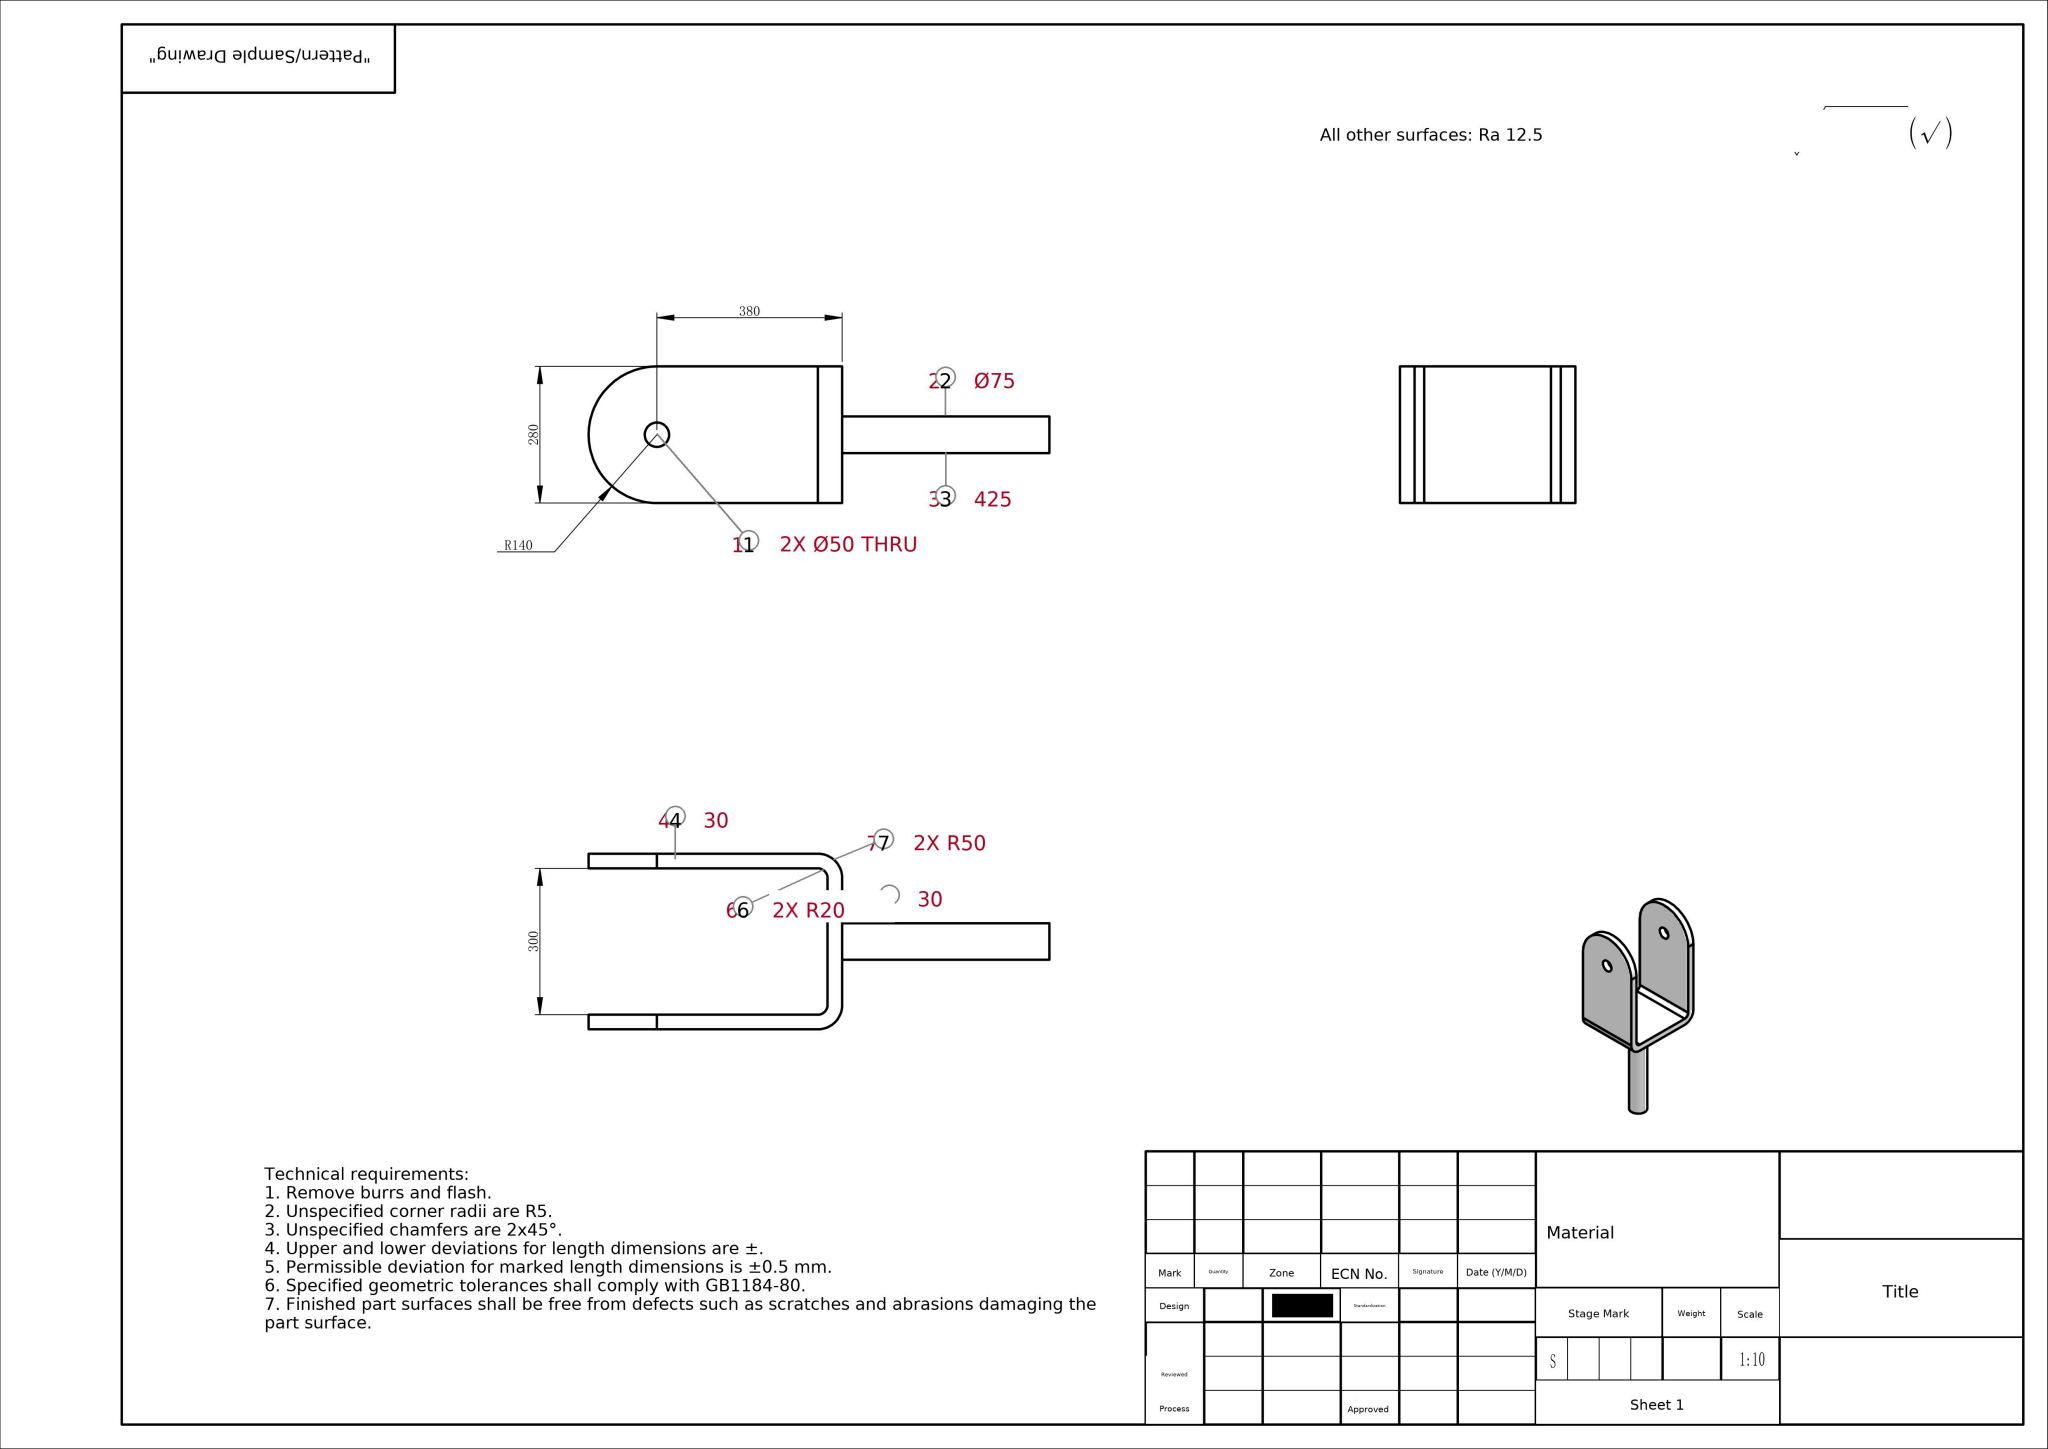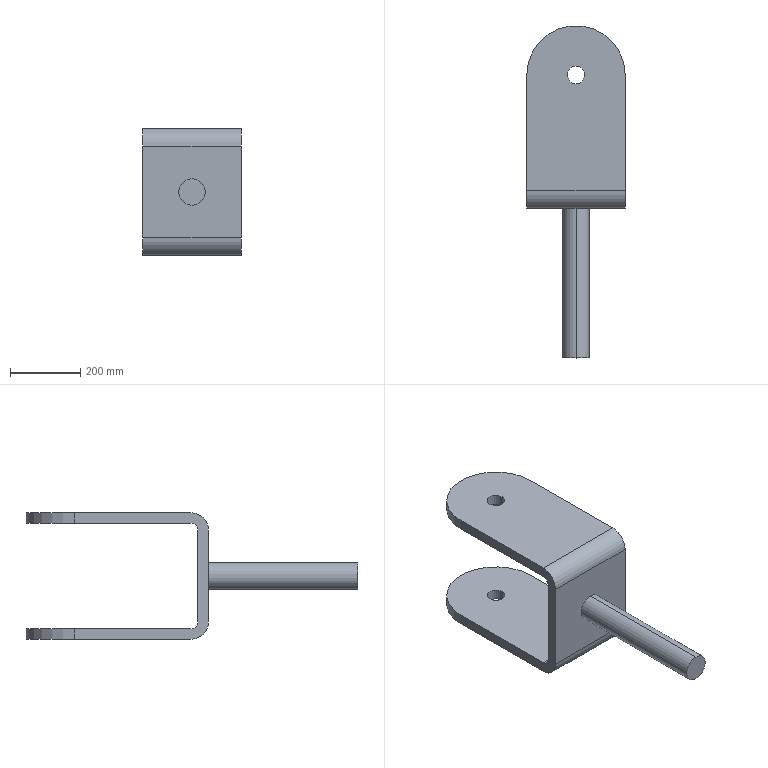Part | SolidWorks | mm | 1 solid | 21 faces | box 280 x 945 x 360 mm | volume 12258667 mm3 | cylinder 12 | plane 9 | commonest cylinder face diameters 50 x4 75 x2 280 x2 40 x2 100 x2
build123d program:
from build123d import *

# Parameters (mm, degrees)
SKETCH1_R           = 25
BOSS_EXTRUDE1_DEPTH = 360
SKETCH2_W           = 300
SKETCH2_H           = 490
CUT_EXTRUDE2_DEPTH  = 360
FILLET1_R           = 20
FILLET2_R           = 50
SKETCH3_R           = 37.5
BOSS_EXTRUDE2_DEPTH = 425


with BuildPart() as part:
    # Sketch1 → Boss-Extrude1 (new body)
    with BuildSketch(Plane.XY):
        with BuildLine():
            Line((-140, 0), (-140, -380))
            Line((-140, -380), (140, -380))
            Line((140, -380), (140, 0))
            ThreePointArc((140, 0), (0, 140), (-140, 0))
        make_face()
        with Locations(Location((0, 0, 0), (0, 0, 180))):
            Circle(SKETCH1_R, mode=Mode.SUBTRACT)
    extrude(amount=BOSS_EXTRUDE1_DEPTH)

    # Sketch2 → Cut-Extrude2 (cut)
    with BuildSketch(Plane(origin=(140, 0, 0), x_dir=(0, 0, -1), z_dir=(1, 0, 0))):
        with Locations((-180, -105)):
            Rectangle(SKETCH2_W, SKETCH2_H)
    extrude(amount=-CUT_EXTRUDE2_DEPTH, mode=Mode.SUBTRACT)

    # Fillet1
    fillet1_edges = [part.edges().sort_by_distance(p)[0] for p in [
        (0, -350, 30),
        (0, -350, 330),
    ]]
    fillet(fillet1_edges, radius=FILLET1_R)

    # Fillet2
    fillet2_edges = [part.edges().sort_by_distance(p)[0] for p in [
        (0, -380, 360),
        (0, -380, 0),
    ]]
    fillet(fillet2_edges, radius=FILLET2_R)

    # Sketch3 → Boss-Extrude2 (add)
    with BuildSketch(Plane.XZ.offset(380)):
        with Locations(Location((0, 180, 0), (0, 0, 90))):
            Circle(SKETCH3_R)
    extrude(amount=BOSS_EXTRUDE2_DEPTH)


solid = part.part
STEP:
#1=CARTESIAN_POINT('',(0.,-805.,142.5));
#2=VERTEX_POINT('',#1);
#3=CARTESIAN_POINT('',(0.,-805.,217.5));
#4=VERTEX_POINT('',#3);
#5=CARTESIAN_POINT('',(0.,-805.,180.));
#6=DIRECTION('',(0.,-1.,0.));
#7=DIRECTION('',(0.,0.,-1.));
#8=AXIS2_PLACEMENT_3D('',#5,#6,#7);
#9=CIRCLE('',#8,37.5);
#10=EDGE_CURVE('',#2,#4,#9,.T.);
#11=ORIENTED_EDGE('',*,*,#10,.F.);
#12=CARTESIAN_POINT('',(0.,-380.,142.5));
#13=VERTEX_POINT('',#12);
#14=CARTESIAN_POINT('',(0.,-805.,142.5));
#15=DIRECTION('',(0.,1.,0.));
#16=VECTOR('',#15,1000.);
#17=LINE('',#14,#16);
#18=EDGE_CURVE('',#2,#13,#17,.T.);
#19=ORIENTED_EDGE('',*,*,#18,.T.);
#20=CARTESIAN_POINT('',(0.,-380.,217.5));
#21=VERTEX_POINT('',#20);
#22=CARTESIAN_POINT('',(0.,-380.,180.));
#23=DIRECTION('',(0.,-1.,0.));
#24=DIRECTION('',(0.,0.,1.));
#25=AXIS2_PLACEMENT_3D('',#22,#23,#24);
#26=CIRCLE('',#25,37.5);
#27=EDGE_CURVE('',#13,#21,#26,.T.);
#28=ORIENTED_EDGE('',*,*,#27,.T.);
#29=CARTESIAN_POINT('',(0.,-805.,217.5));
#30=DIRECTION('',(0.,1.,0.));
#31=VECTOR('',#30,1000.);
#32=LINE('',#29,#31);
#33=EDGE_CURVE('',#4,#21,#32,.T.);
#34=ORIENTED_EDGE('',*,*,#33,.F.);
#35=EDGE_LOOP('',(#11,#19,#28,#34));
#36=FACE_OUTER_BOUND('',#35,.T.);
#37=CARTESIAN_POINT('',(0.,-805.,180.));
#38=DIRECTION('',(0.,1.,0.));
#39=DIRECTION('',(0.,0.,1.));
#40=AXIS2_PLACEMENT_3D('',#37,#38,#39);
#41=CYLINDRICAL_SURFACE('',#40,37.5);
#42=ADVANCED_FACE('',(#36),#41,.T.);
#43=CARTESIAN_POINT('',(-25.,0.,360.));
#44=VERTEX_POINT('',#43);
#45=CARTESIAN_POINT('',(25.,0.,360.));
#46=VERTEX_POINT('',#45);
#47=CARTESIAN_POINT('',(0.,0.,360.));
#48=DIRECTION('',(0.,0.,1.));
#49=DIRECTION('',(1.,0.,0.));
#50=AXIS2_PLACEMENT_3D('',#47,#48,#49);
#51=CIRCLE('',#50,25.);
#52=EDGE_CURVE('',#44,#46,#51,.T.);
#53=ORIENTED_EDGE('',*,*,#52,.T.);
#54=CARTESIAN_POINT('',(25.,0.,330.));
#55=VERTEX_POINT('',#54);
#56=CARTESIAN_POINT('',(25.,0.,360.));
#57=DIRECTION('',(0.,0.,-1.));
#58=VECTOR('',#57,1000.);
#59=LINE('',#56,#58);
#60=EDGE_CURVE('',#46,#55,#59,.T.);
#61=ORIENTED_EDGE('',*,*,#60,.T.);
#62=CARTESIAN_POINT('',(-25.,0.,330.));
#63=VERTEX_POINT('',#62);
#64=CARTESIAN_POINT('',(0.,0.,330.));
#65=DIRECTION('',(-0.,-0.,1.));
#66=DIRECTION('',(0.,-1.,0.));
#67=AXIS2_PLACEMENT_3D('',#64,#65,#66);
#68=CIRCLE('',#67,25.);
#69=EDGE_CURVE('',#63,#55,#68,.T.);
#70=ORIENTED_EDGE('',*,*,#69,.F.);
#71=CARTESIAN_POINT('',(-25.,0.,360.));
#72=DIRECTION('',(0.,0.,-1.));
#73=VECTOR('',#72,1000.);
#74=LINE('',#71,#73);
#75=EDGE_CURVE('',#44,#63,#74,.T.);
#76=ORIENTED_EDGE('',*,*,#75,.F.);
#77=EDGE_LOOP('',(#53,#61,#70,#76));
#78=FACE_OUTER_BOUND('',#77,.T.);
#79=CARTESIAN_POINT('',(0.,0.,360.));
#80=DIRECTION('',(0.,0.,-1.));
#81=DIRECTION('',(-1.,0.,0.));
#82=AXIS2_PLACEMENT_3D('',#79,#80,#81);
#83=CYLINDRICAL_SURFACE('',#82,25.);
#84=ADVANCED_FACE('',(#78),#83,.F.);
#85=CARTESIAN_POINT('',(25.,0.,30.));
#86=VERTEX_POINT('',#85);
#87=CARTESIAN_POINT('',(-25.,0.,30.));
#88=VERTEX_POINT('',#87);
#89=CARTESIAN_POINT('',(0.,0.,30.));
#90=DIRECTION('',(-0.,-0.,-1.));
#91=DIRECTION('',(0.,1.,0.));
#92=AXIS2_PLACEMENT_3D('',#89,#90,#91);
#93=CIRCLE('',#92,25.);
#94=EDGE_CURVE('',#86,#88,#93,.T.);
#95=ORIENTED_EDGE('',*,*,#94,.F.);
#96=CARTESIAN_POINT('',(25.,0.,0.));
#97=VERTEX_POINT('',#96);
#98=CARTESIAN_POINT('',(25.,0.,360.));
#99=DIRECTION('',(0.,0.,-1.));
#100=VECTOR('',#99,1000.);
#101=LINE('',#98,#100);
#102=EDGE_CURVE('',#86,#97,#101,.T.);
#103=ORIENTED_EDGE('',*,*,#102,.T.);
#104=CARTESIAN_POINT('',(-25.,0.,0.));
#105=VERTEX_POINT('',#104);
#106=CARTESIAN_POINT('',(0.,0.,0.));
#107=DIRECTION('',(0.,0.,1.));
#108=DIRECTION('',(1.,0.,0.));
#109=AXIS2_PLACEMENT_3D('',#106,#107,#108);
#110=CIRCLE('',#109,25.);
#111=EDGE_CURVE('',#105,#97,#110,.T.);
#112=ORIENTED_EDGE('',*,*,#111,.F.);
#113=CARTESIAN_POINT('',(-25.,0.,360.));
#114=DIRECTION('',(0.,0.,-1.));
#115=VECTOR('',#114,1000.);
#116=LINE('',#113,#115);
#117=EDGE_CURVE('',#88,#105,#116,.T.);
#118=ORIENTED_EDGE('',*,*,#117,.F.);
#119=EDGE_LOOP('',(#95,#103,#112,#118));
#120=FACE_OUTER_BOUND('',#119,.T.);
#121=CARTESIAN_POINT('',(0.,0.,360.));
#122=DIRECTION('',(0.,0.,-1.));
#123=DIRECTION('',(-1.,0.,0.));
#124=AXIS2_PLACEMENT_3D('',#121,#122,#123);
#125=CYLINDRICAL_SURFACE('',#124,25.);
#126=ADVANCED_FACE('',(#120),#125,.F.);
#127=CARTESIAN_POINT('',(-140.,-0.,30.));
#128=VERTEX_POINT('',#127);
#129=CARTESIAN_POINT('',(140.,0.,30.));
#130=VERTEX_POINT('',#129);
#131=CARTESIAN_POINT('',(0.,0.,30.));
#132=DIRECTION('',(-0.,-0.,-1.));
#133=DIRECTION('',(0.,1.,-0.));
#134=AXIS2_PLACEMENT_3D('',#131,#132,#133);
#135=CIRCLE('',#134,140.);
#136=EDGE_CURVE('',#128,#130,#135,.T.);
#137=ORIENTED_EDGE('',*,*,#136,.T.);
#138=CARTESIAN_POINT('',(140.,0.,0.));
#139=VERTEX_POINT('',#138);
#140=CARTESIAN_POINT('',(140.,0.,360.));
#141=DIRECTION('',(0.,0.,-1.));
#142=VECTOR('',#141,1000.);
#143=LINE('',#140,#142);
#144=EDGE_CURVE('',#130,#139,#143,.T.);
#145=ORIENTED_EDGE('',*,*,#144,.T.);
#146=CARTESIAN_POINT('',(-140.,0.,0.));
#147=VERTEX_POINT('',#146);
#148=CARTESIAN_POINT('',(0.,0.,0.));
#149=DIRECTION('',(0.,0.,1.));
#150=DIRECTION('',(1.,0.,0.));
#151=AXIS2_PLACEMENT_3D('',#148,#149,#150);
#152=CIRCLE('',#151,140.);
#153=EDGE_CURVE('',#139,#147,#152,.T.);
#154=ORIENTED_EDGE('',*,*,#153,.T.);
#155=CARTESIAN_POINT('',(-140.,0.,360.));
#156=DIRECTION('',(0.,0.,-1.));
#157=VECTOR('',#156,1000.);
#158=LINE('',#155,#157);
#159=EDGE_CURVE('',#128,#147,#158,.T.);
#160=ORIENTED_EDGE('',*,*,#159,.F.);
#161=EDGE_LOOP('',(#137,#145,#154,#160));
#162=FACE_OUTER_BOUND('',#161,.T.);
#163=CARTESIAN_POINT('',(0.,0.,360.));
#164=DIRECTION('',(0.,0.,-1.));
#165=DIRECTION('',(-1.,0.,0.));
#166=AXIS2_PLACEMENT_3D('',#163,#164,#165);
#167=CYLINDRICAL_SURFACE('',#166,140.);
#168=ADVANCED_FACE('',(#162),#167,.T.);
#169=ORIENTED_EDGE('',*,*,#102,.F.);
#170=CARTESIAN_POINT('',(0.,0.,30.));
#171=DIRECTION('',(-0.,-0.,-1.));
#172=DIRECTION('',(0.,1.,0.));
#173=AXIS2_PLACEMENT_3D('',#170,#171,#172);
#174=CIRCLE('',#173,25.);
#175=EDGE_CURVE('',#88,#86,#174,.T.);
#176=ORIENTED_EDGE('',*,*,#175,.F.);
#177=ORIENTED_EDGE('',*,*,#117,.T.);
#178=CARTESIAN_POINT('',(0.,0.,0.));
#179=DIRECTION('',(0.,0.,1.));
#180=DIRECTION('',(1.,0.,0.));
#181=AXIS2_PLACEMENT_3D('',#178,#179,#180);
#182=CIRCLE('',#181,25.);
#183=EDGE_CURVE('',#97,#105,#182,.T.);
#184=ORIENTED_EDGE('',*,*,#183,.F.);
#185=EDGE_LOOP('',(#169,#176,#177,#184));
#186=FACE_OUTER_BOUND('',#185,.T.);
#187=CARTESIAN_POINT('',(0.,0.,360.));
#188=DIRECTION('',(0.,0.,-1.));
#189=DIRECTION('',(-1.,0.,0.));
#190=AXIS2_PLACEMENT_3D('',#187,#188,#189);
#191=CYLINDRICAL_SURFACE('',#190,25.);
#192=ADVANCED_FACE('',(#186),#191,.F.);
#193=CARTESIAN_POINT('',(-140.,0.,360.));
#194=VERTEX_POINT('',#193);
#195=CARTESIAN_POINT('',(-140.,-330.,360.));
#196=VERTEX_POINT('',#195);
#197=CARTESIAN_POINT('',(-140.,0.,360.));
#198=DIRECTION('',(0.,-1.,0.));
#199=VECTOR('',#198,1000.);
#200=LINE('',#197,#199);
#201=EDGE_CURVE('',#194,#196,#200,.T.);
#202=ORIENTED_EDGE('',*,*,#201,.T.);
#203=CARTESIAN_POINT('',(140.,-330.,360.));
#204=VERTEX_POINT('',#203);
#205=CARTESIAN_POINT('',(140.,-330.,360.));
#206=DIRECTION('',(1.,0.,0.));
#207=VECTOR('',#206,1000.);
#208=LINE('',#205,#207);
#209=EDGE_CURVE('',#196,#204,#208,.T.);
#210=ORIENTED_EDGE('',*,*,#209,.T.);
#211=CARTESIAN_POINT('',(140.,0.,360.));
#212=VERTEX_POINT('',#211);
#213=CARTESIAN_POINT('',(140.,-380.,360.));
#214=DIRECTION('',(0.,1.,0.));
#215=VECTOR('',#214,1000.);
#216=LINE('',#213,#215);
#217=EDGE_CURVE('',#204,#212,#216,.T.);
#218=ORIENTED_EDGE('',*,*,#217,.T.);
#219=CARTESIAN_POINT('',(0.,0.,360.));
#220=DIRECTION('',(0.,0.,1.));
#221=DIRECTION('',(1.,0.,0.));
#222=AXIS2_PLACEMENT_3D('',#219,#220,#221);
#223=CIRCLE('',#222,140.);
#224=EDGE_CURVE('',#212,#194,#223,.T.);
#225=ORIENTED_EDGE('',*,*,#224,.T.);
#226=EDGE_LOOP('',(#202,#210,#218,#225));
#227=FACE_OUTER_BOUND('',#226,.T.);
#228=ORIENTED_EDGE('',*,*,#52,.F.);
#229=CARTESIAN_POINT('',(0.,0.,360.));
#230=DIRECTION('',(0.,0.,1.));
#231=DIRECTION('',(1.,0.,0.));
#232=AXIS2_PLACEMENT_3D('',#229,#230,#231);
#233=CIRCLE('',#232,25.);
#234=EDGE_CURVE('',#46,#44,#233,.T.);
#235=ORIENTED_EDGE('',*,*,#234,.F.);
#236=EDGE_LOOP('',(#228,#235));
#237=FACE_BOUND('',#236,.T.);
#238=CARTESIAN_POINT('',(0.,0.,360.));
#239=DIRECTION('',(0.,0.,1.));
#240=DIRECTION('',(1.,0.,0.));
#241=AXIS2_PLACEMENT_3D('',#238,#239,#240);
#242=PLANE('',#241);
#243=ADVANCED_FACE('',(#227,#237),#242,.T.);
#244=CARTESIAN_POINT('',(140.,-330.,0.));
#245=VERTEX_POINT('',#244);
#246=CARTESIAN_POINT('',(140.,-380.,0.));
#247=DIRECTION('',(0.,1.,0.));
#248=VECTOR('',#247,1000.);
#249=LINE('',#246,#248);
#250=EDGE_CURVE('',#245,#139,#249,.T.);
#251=ORIENTED_EDGE('',*,*,#250,.F.);
#252=CARTESIAN_POINT('',(-140.,-330.,0.));
#253=VERTEX_POINT('',#252);
#254=CARTESIAN_POINT('',(0.,-330.,0.));
#255=DIRECTION('',(-1.,0.,0.));
#256=VECTOR('',#255,1000.);
#257=LINE('',#254,#256);
#258=EDGE_CURVE('',#245,#253,#257,.T.);
#259=ORIENTED_EDGE('',*,*,#258,.T.);
#260=CARTESIAN_POINT('',(-140.,0.,0.));
#261=DIRECTION('',(0.,-1.,0.));
#262=VECTOR('',#261,1000.);
#263=LINE('',#260,#262);
#264=EDGE_CURVE('',#147,#253,#263,.T.);
#265=ORIENTED_EDGE('',*,*,#264,.F.);
#266=ORIENTED_EDGE('',*,*,#153,.F.);
#267=EDGE_LOOP('',(#251,#259,#265,#266));
#268=FACE_OUTER_BOUND('',#267,.T.);
#269=ORIENTED_EDGE('',*,*,#111,.T.);
#270=ORIENTED_EDGE('',*,*,#183,.T.);
#271=EDGE_LOOP('',(#269,#270));
#272=FACE_BOUND('',#271,.T.);
#273=CARTESIAN_POINT('',(0.,0.,0.));
#274=DIRECTION('',(0.,0.,1.));
#275=DIRECTION('',(1.,0.,0.));
#276=AXIS2_PLACEMENT_3D('',#273,#274,#275);
#277=PLANE('',#276);
#278=ADVANCED_FACE('',(#268,#272),#277,.F.);
#279=CARTESIAN_POINT('',(140.,0.,330.));
#280=VERTEX_POINT('',#279);
#281=CARTESIAN_POINT('',(140.,0.,360.));
#282=DIRECTION('',(0.,0.,-1.));
#283=VECTOR('',#282,1000.);
#284=LINE('',#281,#283);
#285=EDGE_CURVE('',#212,#280,#284,.T.);
#286=ORIENTED_EDGE('',*,*,#285,.T.);
#287=CARTESIAN_POINT('',(-140.,0.,330.));
#288=VERTEX_POINT('',#287);
#289=CARTESIAN_POINT('',(0.,0.,330.));
#290=DIRECTION('',(-0.,-0.,1.));
#291=DIRECTION('',(0.,-1.,0.));
#292=AXIS2_PLACEMENT_3D('',#289,#290,#291);
#293=CIRCLE('',#292,140.);
#294=EDGE_CURVE('',#280,#288,#293,.T.);
#295=ORIENTED_EDGE('',*,*,#294,.T.);
#296=CARTESIAN_POINT('',(-140.,0.,360.));
#297=DIRECTION('',(0.,0.,-1.));
#298=VECTOR('',#297,1000.);
#299=LINE('',#296,#298);
#300=EDGE_CURVE('',#194,#288,#299,.T.);
#301=ORIENTED_EDGE('',*,*,#300,.F.);
#302=ORIENTED_EDGE('',*,*,#224,.F.);
#303=EDGE_LOOP('',(#286,#295,#301,#302));
#304=FACE_OUTER_BOUND('',#303,.T.);
#305=CARTESIAN_POINT('',(0.,0.,360.));
#306=DIRECTION('',(0.,0.,-1.));
#307=DIRECTION('',(-1.,0.,0.));
#308=AXIS2_PLACEMENT_3D('',#305,#306,#307);
#309=CYLINDRICAL_SURFACE('',#308,140.);
#310=ADVANCED_FACE('',(#304),#309,.T.);
#311=ORIENTED_EDGE('',*,*,#264,.T.);
#312=CARTESIAN_POINT('',(-140.,-380.,50.));
#313=VERTEX_POINT('',#312);
#314=CARTESIAN_POINT('',(-140.,-330.,50.));
#315=DIRECTION('',(-1.,-0.,0.));
#316=DIRECTION('',(0.,1.,0.));
#317=AXIS2_PLACEMENT_3D('',#314,#315,#316);
#318=CIRCLE('',#317,50.);
#319=EDGE_CURVE('',#253,#313,#318,.T.);
#320=ORIENTED_EDGE('',*,*,#319,.T.);
#321=CARTESIAN_POINT('',(-140.,-380.,310.));
#322=VERTEX_POINT('',#321);
#323=CARTESIAN_POINT('',(-140.,-380.,360.));
#324=DIRECTION('',(0.,0.,-1.));
#325=VECTOR('',#324,1000.);
#326=LINE('',#323,#325);
#327=EDGE_CURVE('',#322,#313,#326,.T.);
#328=ORIENTED_EDGE('',*,*,#327,.F.);
#329=CARTESIAN_POINT('',(-140.,-330.,310.));
#330=DIRECTION('',(-1.,-0.,0.));
#331=DIRECTION('',(0.,1.,0.));
#332=AXIS2_PLACEMENT_3D('',#329,#330,#331);
#333=CIRCLE('',#332,50.);
#334=EDGE_CURVE('',#322,#196,#333,.T.);
#335=ORIENTED_EDGE('',*,*,#334,.T.);
#336=ORIENTED_EDGE('',*,*,#201,.F.);
#337=ORIENTED_EDGE('',*,*,#300,.T.);
#338=CARTESIAN_POINT('',(-140.,-330.,330.));
#339=VERTEX_POINT('',#338);
#340=CARTESIAN_POINT('',(-140.,0.,330.));
#341=DIRECTION('',(0.,-1.,-0.));
#342=VECTOR('',#341,1000.);
#343=LINE('',#340,#342);
#344=EDGE_CURVE('',#288,#339,#343,.T.);
#345=ORIENTED_EDGE('',*,*,#344,.T.);
#346=CARTESIAN_POINT('',(-140.,-350.,310.));
#347=VERTEX_POINT('',#346);
#348=CARTESIAN_POINT('',(-140.,-330.,310.));
#349=DIRECTION('',(1.,0.,0.));
#350=DIRECTION('',(0.,1.,0.));
#351=AXIS2_PLACEMENT_3D('',#348,#349,#350);
#352=CIRCLE('',#351,20.);
#353=EDGE_CURVE('',#339,#347,#352,.T.);
#354=ORIENTED_EDGE('',*,*,#353,.T.);
#355=CARTESIAN_POINT('',(-140.,-350.,50.));
#356=VERTEX_POINT('',#355);
#357=CARTESIAN_POINT('',(-140.,-350.,360.));
#358=DIRECTION('',(0.,0.,-1.));
#359=VECTOR('',#358,1000.);
#360=LINE('',#357,#359);
#361=EDGE_CURVE('',#347,#356,#360,.T.);
#362=ORIENTED_EDGE('',*,*,#361,.T.);
#363=CARTESIAN_POINT('',(-140.,-330.,30.));
#364=VERTEX_POINT('',#363);
#365=CARTESIAN_POINT('',(-140.,-330.,50.));
#366=DIRECTION('',(1.,0.,0.));
#367=DIRECTION('',(0.,1.,0.));
#368=AXIS2_PLACEMENT_3D('',#365,#366,#367);
#369=CIRCLE('',#368,20.);
#370=EDGE_CURVE('',#356,#364,#369,.T.);
#371=ORIENTED_EDGE('',*,*,#370,.T.);
#372=CARTESIAN_POINT('',(-140.,-0.,30.));
#373=DIRECTION('',(-0.,1.,-0.));
#374=VECTOR('',#373,1000.);
#375=LINE('',#372,#374);
#376=EDGE_CURVE('',#364,#128,#375,.T.);
#377=ORIENTED_EDGE('',*,*,#376,.T.);
#378=ORIENTED_EDGE('',*,*,#159,.T.);
#379=EDGE_LOOP('',(#311,#320,#328,#335,#336,#337,#345,#354,#362,#371,#377,#378));
#380=FACE_OUTER_BOUND('',#379,.T.);
#381=CARTESIAN_POINT('',(-140.,0.,360.));
#382=DIRECTION('',(1.,0.,0.));
#383=DIRECTION('',(-0.,1.,0.));
#384=AXIS2_PLACEMENT_3D('',#381,#382,#383);
#385=PLANE('',#384);
#386=ADVANCED_FACE('',(#380),#385,.F.);
#387=CARTESIAN_POINT('',(0.,-380.,180.));
#388=DIRECTION('',(0.,-1.,0.));
#389=DIRECTION('',(0.,0.,1.));
#390=AXIS2_PLACEMENT_3D('',#387,#388,#389);
#391=CIRCLE('',#390,37.5);
#392=EDGE_CURVE('',#21,#13,#391,.T.);
#393=ORIENTED_EDGE('',*,*,#392,.F.);
#394=ORIENTED_EDGE('',*,*,#27,.F.);
#395=EDGE_LOOP('',(#393,#394));
#396=FACE_BOUND('',#395,.T.);
#397=ORIENTED_EDGE('',*,*,#327,.T.);
#398=CARTESIAN_POINT('',(140.,-380.,50.));
#399=VERTEX_POINT('',#398);
#400=CARTESIAN_POINT('',(-140.,-380.,50.));
#401=DIRECTION('',(1.,0.,0.));
#402=VECTOR('',#401,1000.);
#403=LINE('',#400,#402);
#404=EDGE_CURVE('',#313,#399,#403,.T.);
#405=ORIENTED_EDGE('',*,*,#404,.T.);
#406=CARTESIAN_POINT('',(140.,-380.,310.));
#407=VERTEX_POINT('',#406);
#408=CARTESIAN_POINT('',(140.,-380.,360.));
#409=DIRECTION('',(0.,0.,-1.));
#410=VECTOR('',#409,1000.);
#411=LINE('',#408,#410);
#412=EDGE_CURVE('',#407,#399,#411,.T.);
#413=ORIENTED_EDGE('',*,*,#412,.F.);
#414=CARTESIAN_POINT('',(-140.,-380.,310.));
#415=DIRECTION('',(-1.,0.,0.));
#416=VECTOR('',#415,1000.);
#417=LINE('',#414,#416);
#418=EDGE_CURVE('',#407,#322,#417,.T.);
#419=ORIENTED_EDGE('',*,*,#418,.T.);
#420=EDGE_LOOP('',(#397,#405,#413,#419));
#421=FACE_OUTER_BOUND('',#420,.T.);
#422=CARTESIAN_POINT('',(-140.,-380.,360.));
#423=DIRECTION('',(0.,1.,0.));
#424=DIRECTION('',(0.,0.,1.));
#425=AXIS2_PLACEMENT_3D('',#422,#423,#424);
#426=PLANE('',#425);
#427=ADVANCED_FACE('',(#396,#421),#426,.F.);
#428=ORIENTED_EDGE('',*,*,#412,.T.);
#429=CARTESIAN_POINT('',(140.,-330.,50.));
#430=DIRECTION('',(1.,-0.,0.));
#431=DIRECTION('',(0.,-1.,0.));
#432=AXIS2_PLACEMENT_3D('',#429,#430,#431);
#433=CIRCLE('',#432,50.);
#434=EDGE_CURVE('',#399,#245,#433,.T.);
#435=ORIENTED_EDGE('',*,*,#434,.T.);
#436=ORIENTED_EDGE('',*,*,#250,.T.);
#437=ORIENTED_EDGE('',*,*,#144,.F.);
#438=CARTESIAN_POINT('',(140.,-330.,30.));
#439=VERTEX_POINT('',#438);
#440=CARTESIAN_POINT('',(140.,-350.,30.));
#441=DIRECTION('',(0.,1.,-0.));
#442=VECTOR('',#441,1000.);
#443=LINE('',#440,#442);
#444=EDGE_CURVE('',#439,#130,#443,.T.);
#445=ORIENTED_EDGE('',*,*,#444,.F.);
#446=CARTESIAN_POINT('',(140.,-350.,50.));
#447=VERTEX_POINT('',#446);
#448=CARTESIAN_POINT('',(140.,-330.,50.));
#449=DIRECTION('',(-1.,0.,0.));
#450=DIRECTION('',(0.,-1.,0.));
#451=AXIS2_PLACEMENT_3D('',#448,#449,#450);
#452=CIRCLE('',#451,20.);
#453=EDGE_CURVE('',#439,#447,#452,.T.);
#454=ORIENTED_EDGE('',*,*,#453,.T.);
#455=CARTESIAN_POINT('',(140.,-350.,310.));
#456=VERTEX_POINT('',#455);
#457=CARTESIAN_POINT('',(140.,-350.,330.));
#458=DIRECTION('',(0.,0.,-1.));
#459=VECTOR('',#458,1000.);
#460=LINE('',#457,#459);
#461=EDGE_CURVE('',#456,#447,#460,.T.);
#462=ORIENTED_EDGE('',*,*,#461,.F.);
#463=CARTESIAN_POINT('',(140.,-330.,330.));
#464=VERTEX_POINT('',#463);
#465=CARTESIAN_POINT('',(140.,-330.,310.));
#466=DIRECTION('',(-1.,0.,0.));
#467=DIRECTION('',(0.,-1.,0.));
#468=AXIS2_PLACEMENT_3D('',#465,#466,#467);
#469=CIRCLE('',#468,20.);
#470=EDGE_CURVE('',#456,#464,#469,.T.);
#471=ORIENTED_EDGE('',*,*,#470,.T.);
#472=CARTESIAN_POINT('',(140.,140.,330.));
#473=DIRECTION('',(-0.,-1.,-0.));
#474=VECTOR('',#473,1000.);
#475=LINE('',#472,#474);
#476=EDGE_CURVE('',#280,#464,#475,.T.);
#477=ORIENTED_EDGE('',*,*,#476,.F.);
#478=ORIENTED_EDGE('',*,*,#285,.F.);
#479=ORIENTED_EDGE('',*,*,#217,.F.);
#480=CARTESIAN_POINT('',(140.,-330.,310.));
#481=DIRECTION('',(1.,-0.,0.));
#482=DIRECTION('',(0.,-1.,0.));
#483=AXIS2_PLACEMENT_3D('',#480,#481,#482);
#484=CIRCLE('',#483,50.);
#485=EDGE_CURVE('',#204,#407,#484,.T.);
#486=ORIENTED_EDGE('',*,*,#485,.T.);
#487=EDGE_LOOP('',(#428,#435,#436,#437,#445,#454,#462,#471,#477,#478,#479,#486));
#488=FACE_OUTER_BOUND('',#487,.T.);
#489=CARTESIAN_POINT('',(140.,-380.,360.));
#490=DIRECTION('',(-1.,0.,0.));
#491=DIRECTION('',(-0.,-1.,0.));
#492=AXIS2_PLACEMENT_3D('',#489,#490,#491);
#493=PLANE('',#492);
#494=ADVANCED_FACE('',(#488),#493,.F.);
#495=ORIENTED_EDGE('',*,*,#60,.F.);
#496=ORIENTED_EDGE('',*,*,#234,.T.);
#497=ORIENTED_EDGE('',*,*,#75,.T.);
#498=CARTESIAN_POINT('',(0.,0.,330.));
#499=DIRECTION('',(-0.,-0.,1.));
#500=DIRECTION('',(0.,-1.,0.));
#501=AXIS2_PLACEMENT_3D('',#498,#499,#500);
#502=CIRCLE('',#501,25.);
#503=EDGE_CURVE('',#55,#63,#502,.T.);
#504=ORIENTED_EDGE('',*,*,#503,.F.);
#505=EDGE_LOOP('',(#495,#496,#497,#504));
#506=FACE_OUTER_BOUND('',#505,.T.);
#507=CARTESIAN_POINT('',(0.,0.,360.));
#508=DIRECTION('',(0.,0.,-1.));
#509=DIRECTION('',(-1.,0.,0.));
#510=AXIS2_PLACEMENT_3D('',#507,#508,#509);
#511=CYLINDRICAL_SURFACE('',#510,25.);
#512=ADVANCED_FACE('',(#506),#511,.F.);
#513=ORIENTED_EDGE('',*,*,#461,.T.);
#514=CARTESIAN_POINT('',(-140.,-350.,50.));
#515=DIRECTION('',(-1.,0.,0.));
#516=VECTOR('',#515,1000.);
#517=LINE('',#514,#516);
#518=EDGE_CURVE('',#447,#356,#517,.T.);
#519=ORIENTED_EDGE('',*,*,#518,.T.);
#520=ORIENTED_EDGE('',*,*,#361,.F.);
#521=CARTESIAN_POINT('',(140.,-350.,310.));
#522=DIRECTION('',(1.,-0.,0.));
#523=VECTOR('',#522,1000.);
#524=LINE('',#521,#523);
#525=EDGE_CURVE('',#347,#456,#524,.T.);
#526=ORIENTED_EDGE('',*,*,#525,.T.);
#527=EDGE_LOOP('',(#513,#519,#520,#526));
#528=FACE_OUTER_BOUND('',#527,.T.);
#529=CARTESIAN_POINT('',(-220.,-350.,330.));
#530=DIRECTION('',(-0.,-1.,0.));
#531=DIRECTION('',(1.,-0.,0.));
#532=AXIS2_PLACEMENT_3D('',#529,#530,#531);
#533=PLANE('',#532);
#534=ADVANCED_FACE('',(#528),#533,.F.);
#535=ORIENTED_EDGE('',*,*,#175,.T.);
#536=ORIENTED_EDGE('',*,*,#94,.T.);
#537=EDGE_LOOP('',(#535,#536));
#538=FACE_BOUND('',#537,.T.);
#539=ORIENTED_EDGE('',*,*,#376,.F.);
#540=CARTESIAN_POINT('',(140.,-330.,30.));
#541=DIRECTION('',(1.,-0.,0.));
#542=VECTOR('',#541,1000.);
#543=LINE('',#540,#542);
#544=EDGE_CURVE('',#364,#439,#543,.T.);
#545=ORIENTED_EDGE('',*,*,#544,.T.);
#546=ORIENTED_EDGE('',*,*,#444,.T.);
#547=ORIENTED_EDGE('',*,*,#136,.F.);
#548=EDGE_LOOP('',(#539,#545,#546,#547));
#549=FACE_OUTER_BOUND('',#548,.T.);
#550=CARTESIAN_POINT('',(-220.,-350.,30.));
#551=DIRECTION('',(-0.,-0.,-1.));
#552=DIRECTION('',(0.,1.,-0.));
#553=AXIS2_PLACEMENT_3D('',#550,#551,#552);
#554=PLANE('',#553);
#555=ADVANCED_FACE('',(#538,#549),#554,.F.);
#556=ORIENTED_EDGE('',*,*,#69,.T.);
#557=ORIENTED_EDGE('',*,*,#503,.T.);
#558=EDGE_LOOP('',(#556,#557));
#559=FACE_BOUND('',#558,.T.);
#560=ORIENTED_EDGE('',*,*,#476,.T.);
#561=CARTESIAN_POINT('',(-140.,-330.,330.));
#562=DIRECTION('',(-1.,0.,0.));
#563=VECTOR('',#562,1000.);
#564=LINE('',#561,#563);
#565=EDGE_CURVE('',#464,#339,#564,.T.);
#566=ORIENTED_EDGE('',*,*,#565,.T.);
#567=ORIENTED_EDGE('',*,*,#344,.F.);
#568=ORIENTED_EDGE('',*,*,#294,.F.);
#569=EDGE_LOOP('',(#560,#566,#567,#568));
#570=FACE_OUTER_BOUND('',#569,.T.);
#571=CARTESIAN_POINT('',(-220.,140.,330.));
#572=DIRECTION('',(-0.,-0.,1.));
#573=DIRECTION('',(0.,-1.,-0.));
#574=AXIS2_PLACEMENT_3D('',#571,#572,#573);
#575=PLANE('',#574);
#576=ADVANCED_FACE('',(#559,#570),#575,.F.);
#577=ORIENTED_EDGE('',*,*,#370,.F.);
#578=ORIENTED_EDGE('',*,*,#518,.F.);
#579=ORIENTED_EDGE('',*,*,#453,.F.);
#580=ORIENTED_EDGE('',*,*,#544,.F.);
#581=EDGE_LOOP('',(#577,#578,#579,#580));
#582=FACE_OUTER_BOUND('',#581,.T.);
#583=CARTESIAN_POINT('',(-220.,-330.,50.));
#584=DIRECTION('',(-1.,0.,0.));
#585=DIRECTION('',(0.,-1.,0.));
#586=AXIS2_PLACEMENT_3D('',#583,#584,#585);
#587=CYLINDRICAL_SURFACE('',#586,20.);
#588=ADVANCED_FACE('',(#582),#587,.F.);
#589=ORIENTED_EDGE('',*,*,#353,.F.);
#590=ORIENTED_EDGE('',*,*,#565,.F.);
#591=ORIENTED_EDGE('',*,*,#470,.F.);
#592=ORIENTED_EDGE('',*,*,#525,.F.);
#593=EDGE_LOOP('',(#589,#590,#591,#592));
#594=FACE_OUTER_BOUND('',#593,.T.);
#595=CARTESIAN_POINT('',(-220.,-330.,310.));
#596=DIRECTION('',(-1.,0.,0.));
#597=DIRECTION('',(0.,-1.,0.));
#598=AXIS2_PLACEMENT_3D('',#595,#596,#597);
#599=CYLINDRICAL_SURFACE('',#598,20.);
#600=ADVANCED_FACE('',(#594),#599,.F.);
#601=ORIENTED_EDGE('',*,*,#319,.F.);
#602=ORIENTED_EDGE('',*,*,#258,.F.);
#603=ORIENTED_EDGE('',*,*,#434,.F.);
#604=ORIENTED_EDGE('',*,*,#404,.F.);
#605=EDGE_LOOP('',(#601,#602,#603,#604));
#606=FACE_OUTER_BOUND('',#605,.T.);
#607=CARTESIAN_POINT('',(-140.,-330.,50.));
#608=DIRECTION('',(1.,0.,0.));
#609=DIRECTION('',(0.,0.,-1.));
#610=AXIS2_PLACEMENT_3D('',#607,#608,#609);
#611=CYLINDRICAL_SURFACE('',#610,50.);
#612=ADVANCED_FACE('',(#606),#611,.T.);
#613=ORIENTED_EDGE('',*,*,#334,.F.);
#614=ORIENTED_EDGE('',*,*,#418,.F.);
#615=ORIENTED_EDGE('',*,*,#485,.F.);
#616=ORIENTED_EDGE('',*,*,#209,.F.);
#617=EDGE_LOOP('',(#613,#614,#615,#616));
#618=FACE_OUTER_BOUND('',#617,.T.);
#619=CARTESIAN_POINT('',(0.,-330.,310.));
#620=DIRECTION('',(-1.,0.,0.));
#621=DIRECTION('',(0.,0.,1.));
#622=AXIS2_PLACEMENT_3D('',#619,#620,#621);
#623=CYLINDRICAL_SURFACE('',#622,50.);
#624=ADVANCED_FACE('',(#618),#623,.T.);
#625=ORIENTED_EDGE('',*,*,#18,.F.);
#626=CARTESIAN_POINT('',(0.,-805.,180.));
#627=DIRECTION('',(0.,-1.,0.));
#628=DIRECTION('',(0.,0.,-1.));
#629=AXIS2_PLACEMENT_3D('',#626,#627,#628);
#630=CIRCLE('',#629,37.5);
#631=EDGE_CURVE('',#4,#2,#630,.T.);
#632=ORIENTED_EDGE('',*,*,#631,.F.);
#633=ORIENTED_EDGE('',*,*,#33,.T.);
#634=ORIENTED_EDGE('',*,*,#392,.T.);
#635=EDGE_LOOP('',(#625,#632,#633,#634));
#636=FACE_OUTER_BOUND('',#635,.T.);
#637=CARTESIAN_POINT('',(0.,-805.,180.));
#638=DIRECTION('',(0.,1.,0.));
#639=DIRECTION('',(0.,0.,1.));
#640=AXIS2_PLACEMENT_3D('',#637,#638,#639);
#641=CYLINDRICAL_SURFACE('',#640,37.5);
#642=ADVANCED_FACE('',(#636),#641,.T.);
#643=ORIENTED_EDGE('',*,*,#631,.T.);
#644=ORIENTED_EDGE('',*,*,#10,.T.);
#645=EDGE_LOOP('',(#643,#644));
#646=FACE_OUTER_BOUND('',#645,.T.);
#647=CARTESIAN_POINT('',(0.,-805.,180.));
#648=DIRECTION('',(0.,-1.,0.));
#649=DIRECTION('',(0.,0.,-1.));
#650=AXIS2_PLACEMENT_3D('',#647,#648,#649);
#651=PLANE('',#650);
#652=ADVANCED_FACE('',(#646),#651,.T.);
#653=CLOSED_SHELL('',(#42,#84,#126,#168,#192,#243,#278,#310,#386,#427,#494,#512,#534,#555,#576,#588,#600,#612,#624,#642,#652));
#654=MANIFOLD_SOLID_BREP('',#653);
#655=CARTESIAN_POINT('',(0.,0.,0.));
#656=DIRECTION('',(0.,0.,1.));
#657=DIRECTION('',(1.,0.,0.));
#658=AXIS2_PLACEMENT_3D('',#655,#656,#657);
#659=(LENGTH_UNIT()NAMED_UNIT(*)SI_UNIT(.MILLI.,.METRE.));
#660=UNCERTAINTY_MEASURE_WITH_UNIT(LENGTH_MEASURE(0.00001),#659,'','');
#661=(NAMED_UNIT(*)PLANE_ANGLE_UNIT()SI_UNIT($,.RADIAN.));
#662=(NAMED_UNIT(*)SI_UNIT($,.STERADIAN.)SOLID_ANGLE_UNIT());
#663=(GEOMETRIC_REPRESENTATION_CONTEXT(3)GLOBAL_UNCERTAINTY_ASSIGNED_CONTEXT((#660))GLOBAL_UNIT_ASSIGNED_CONTEXT((#659,#661,#662))REPRESENTATION_CONTEXT('',''));
#664=ADVANCED_BREP_SHAPE_REPRESENTATION('',(#654,#658),#663);